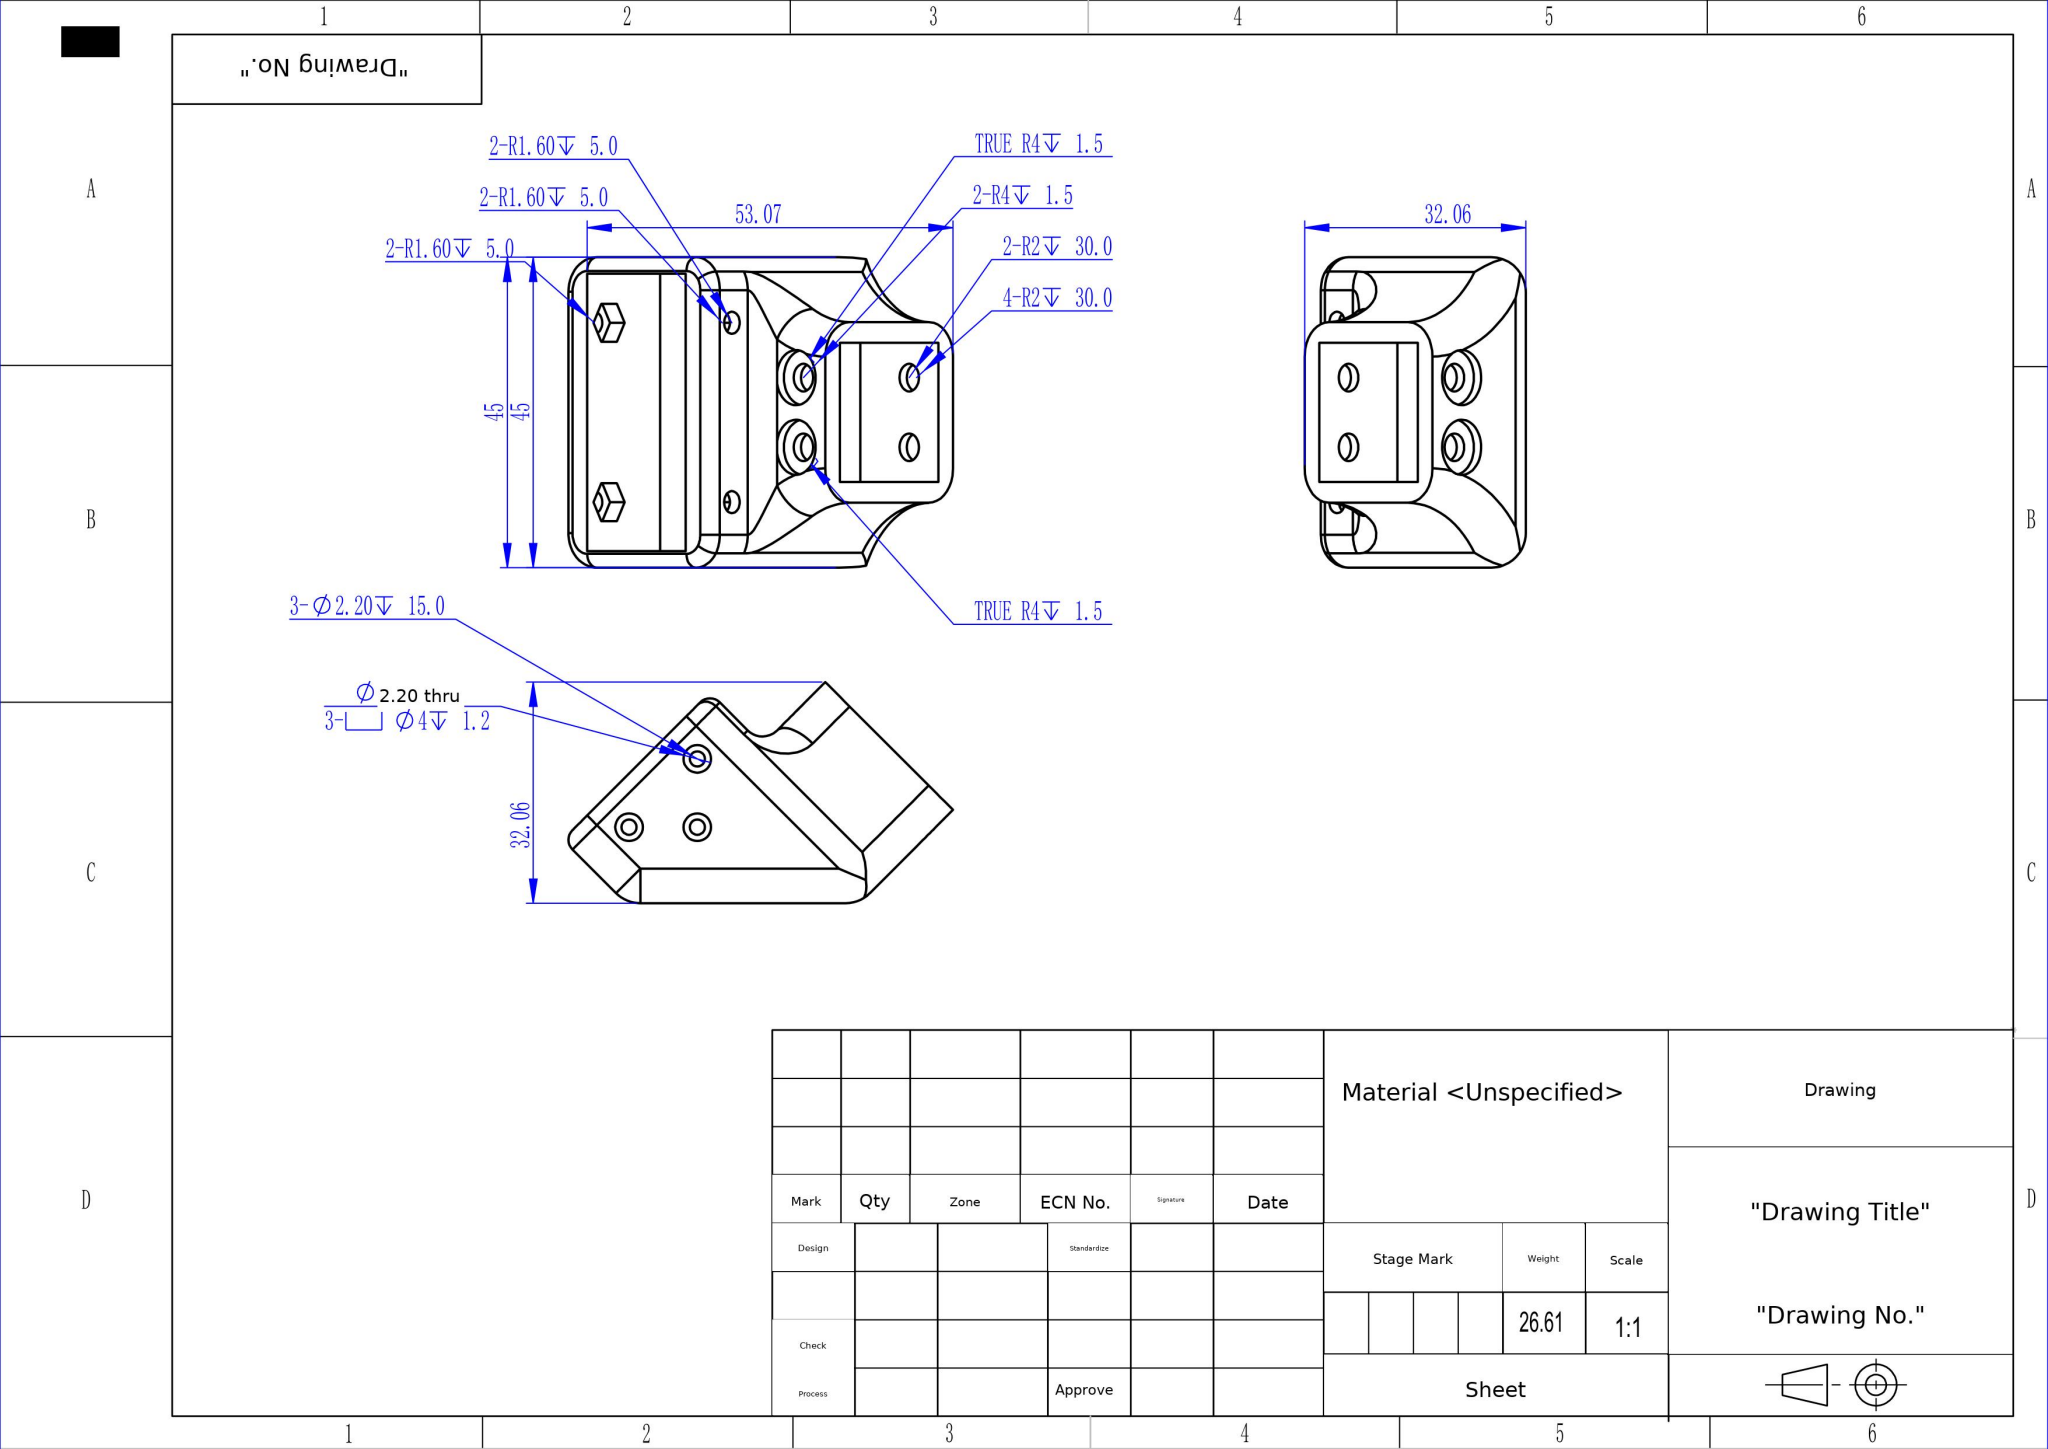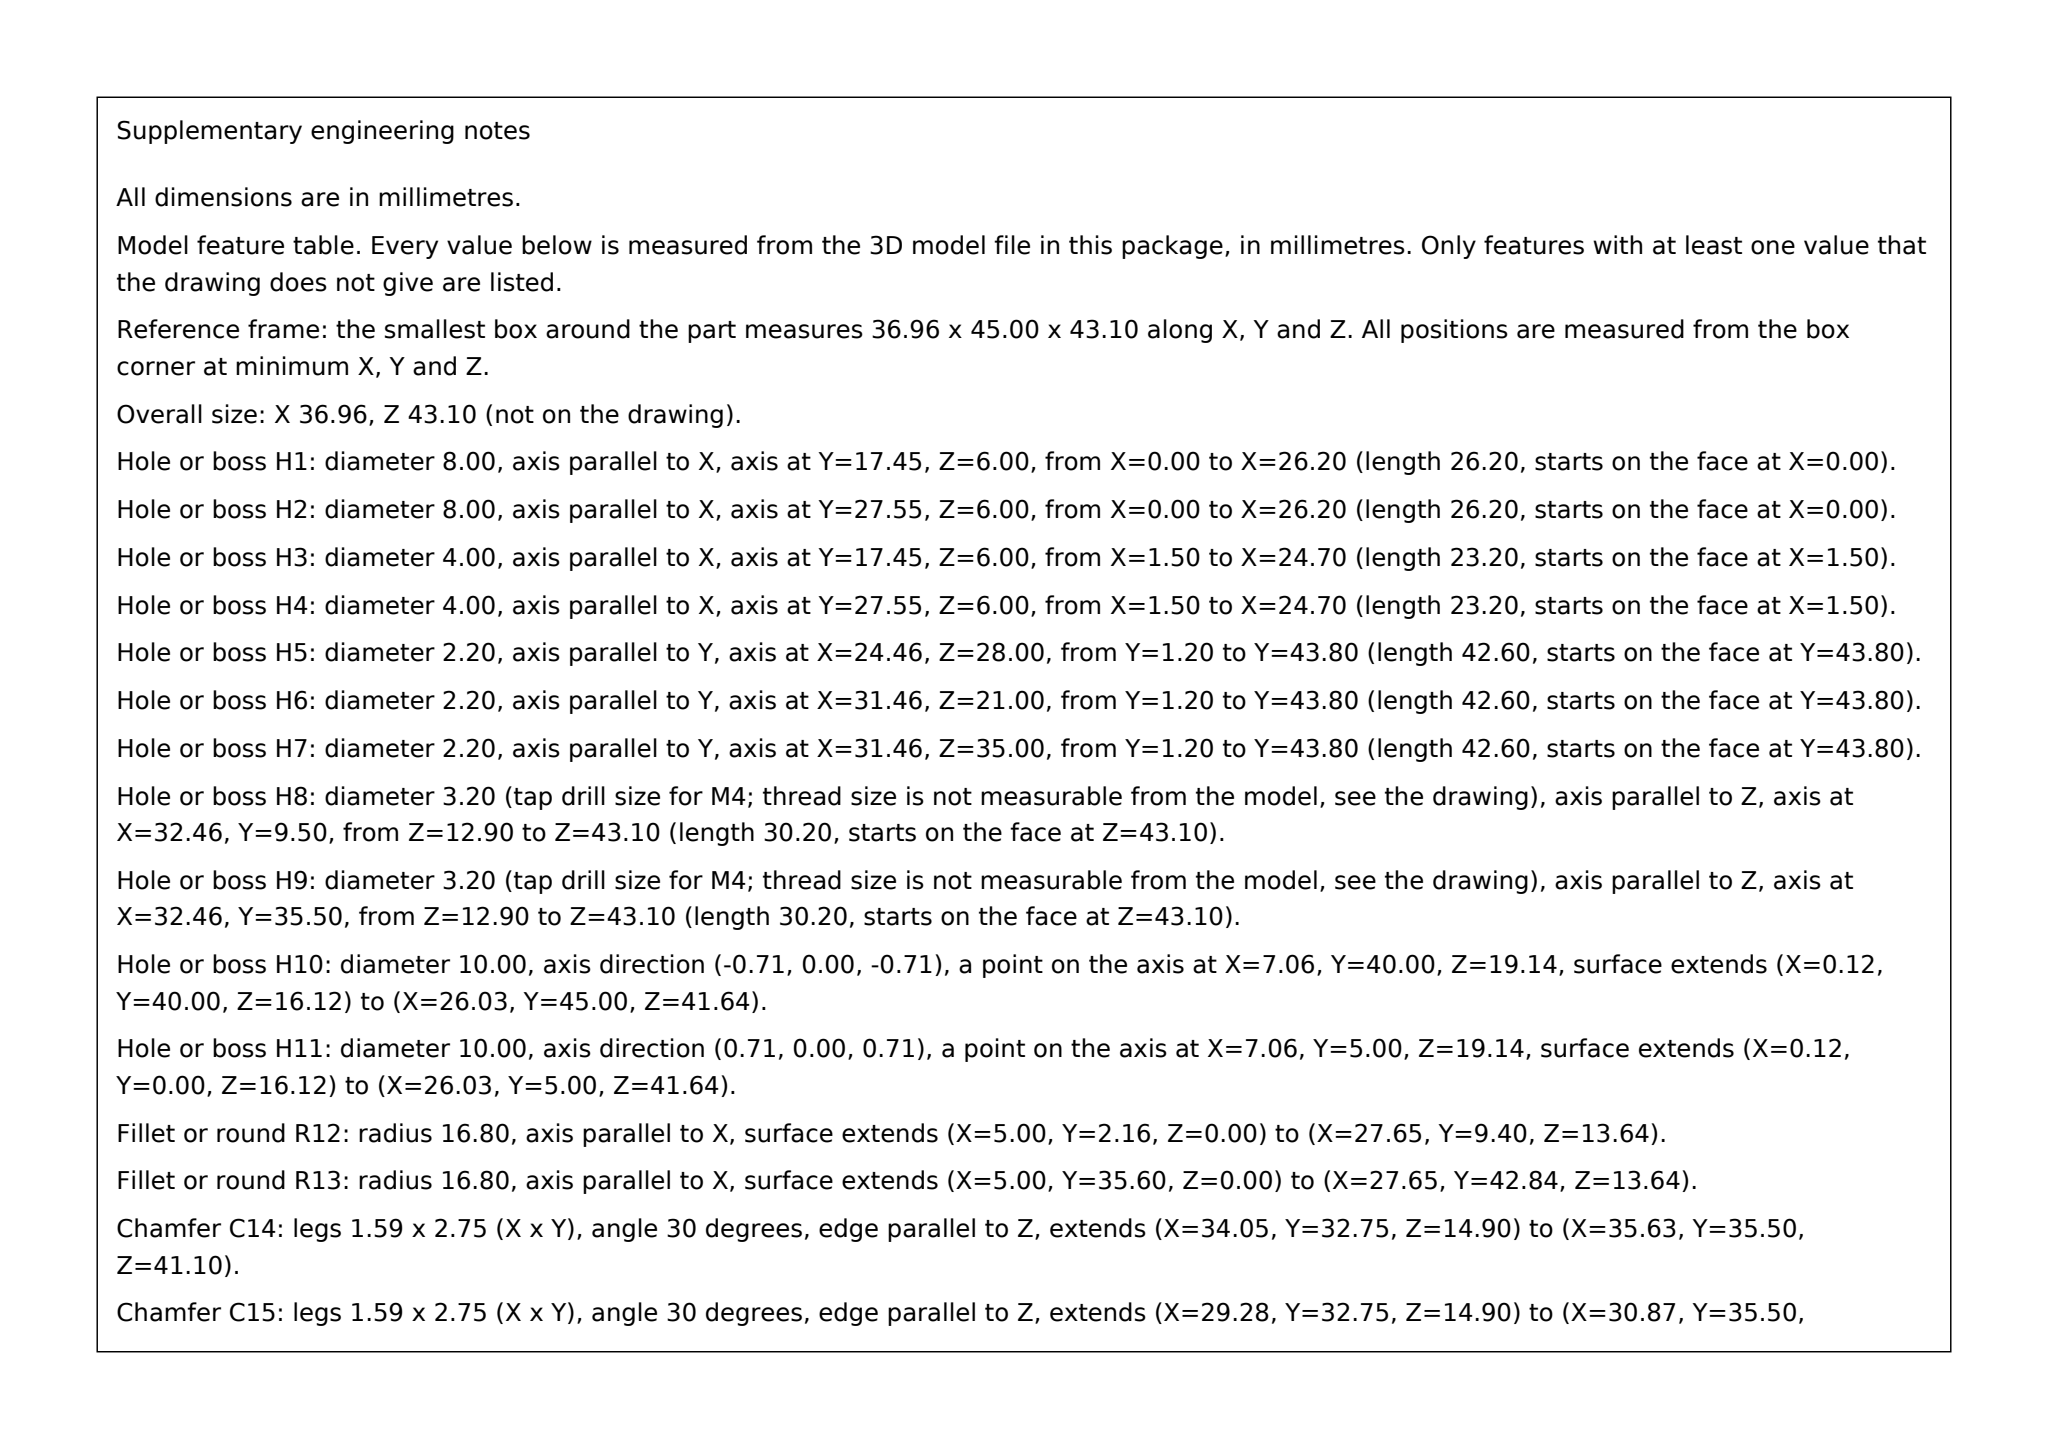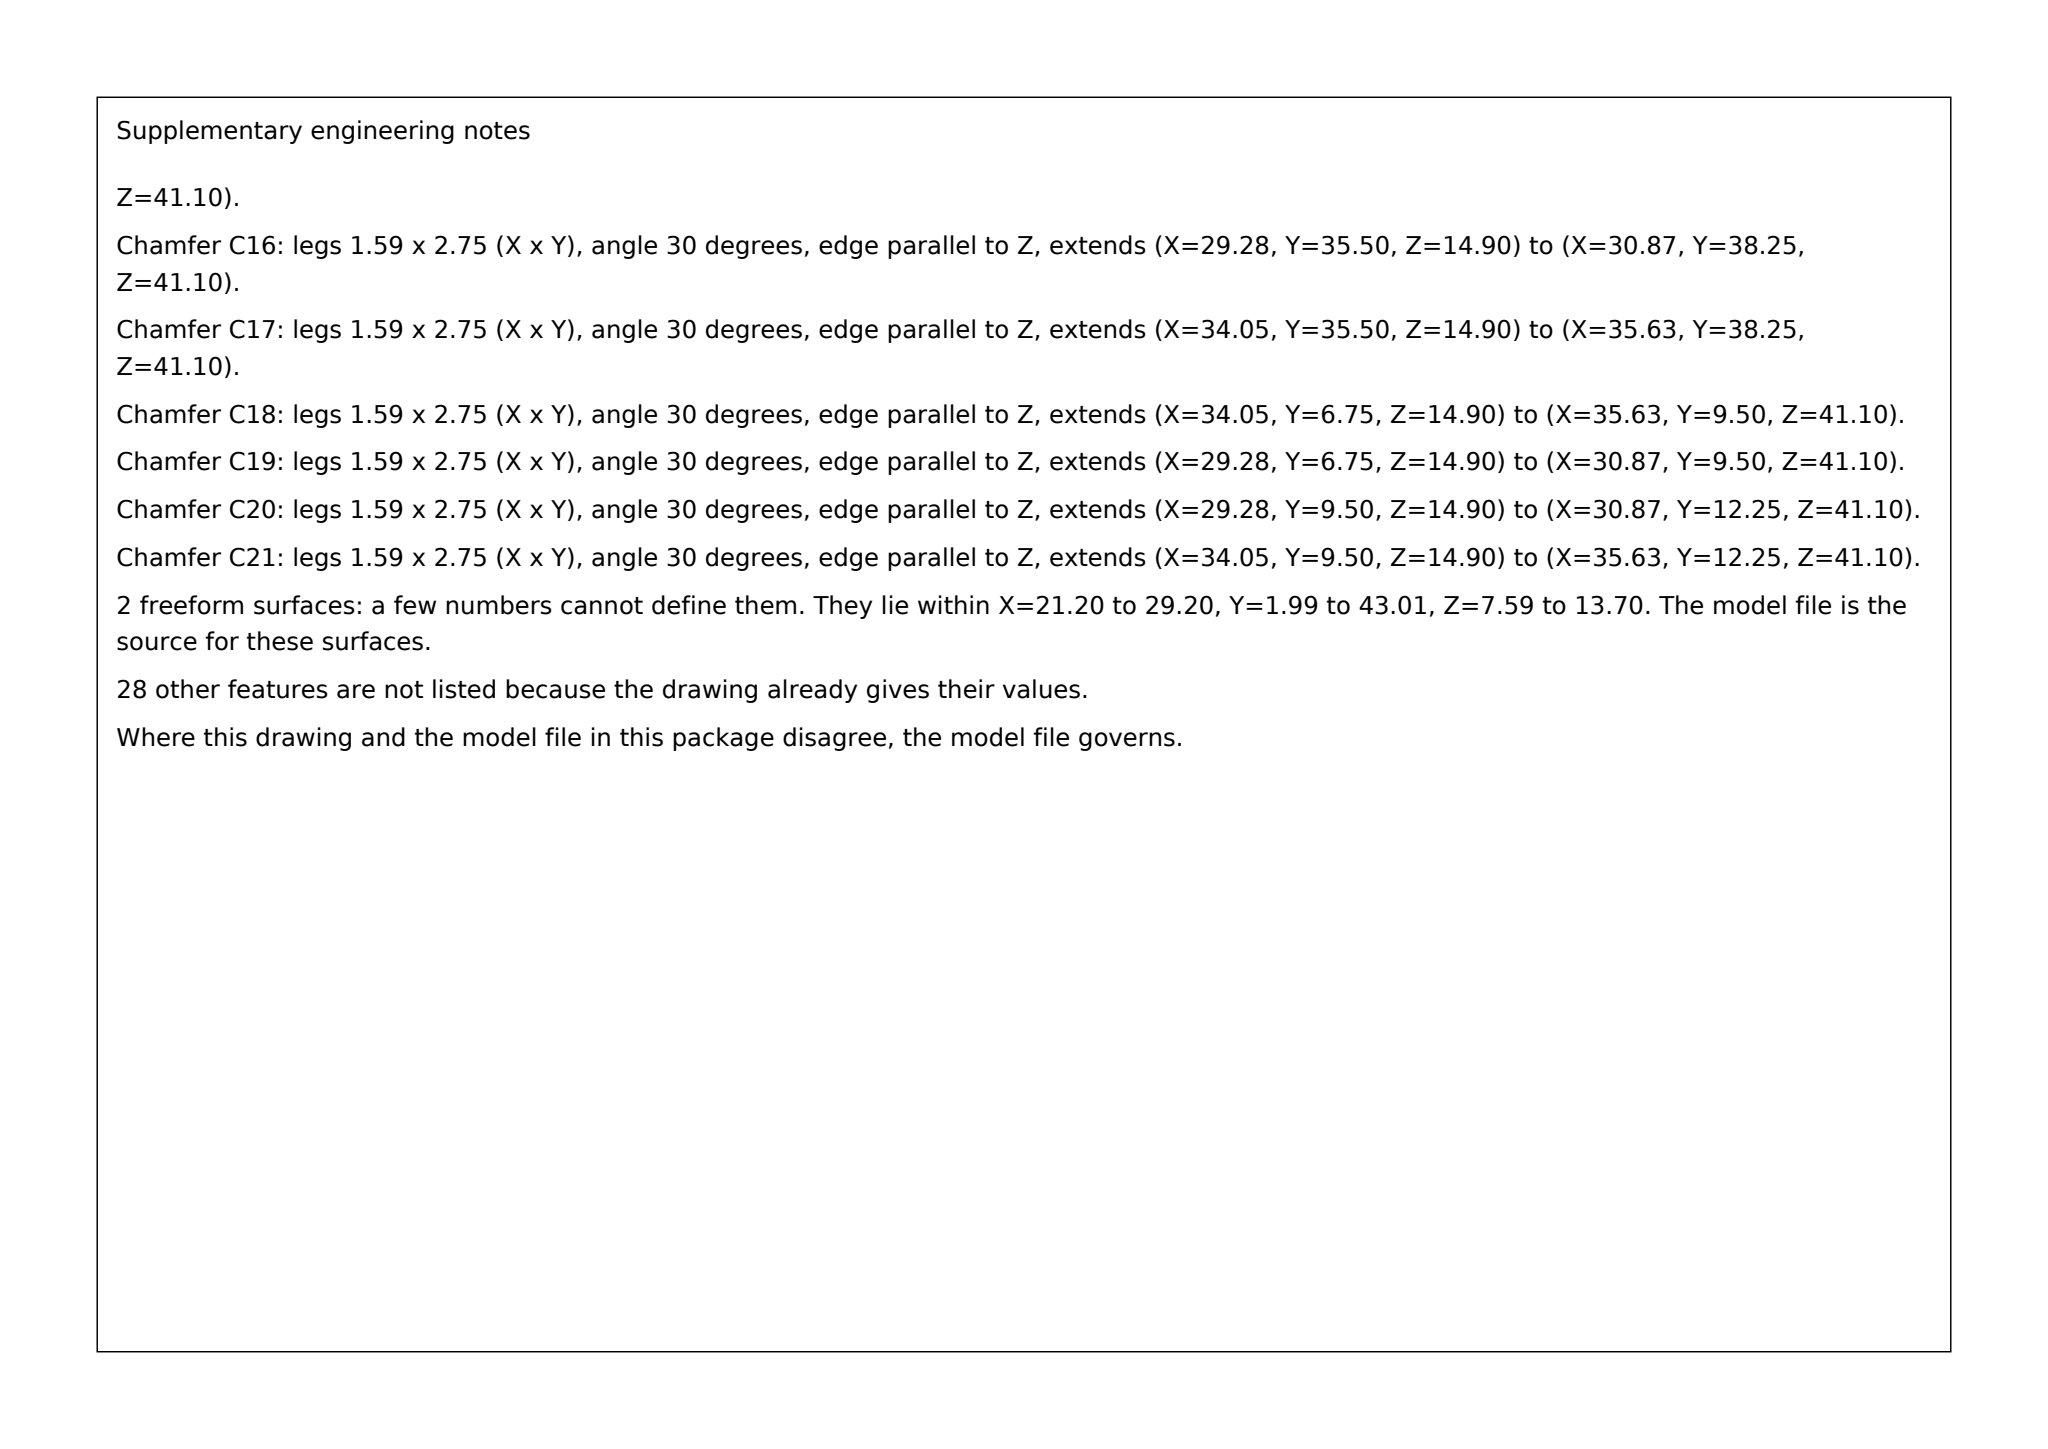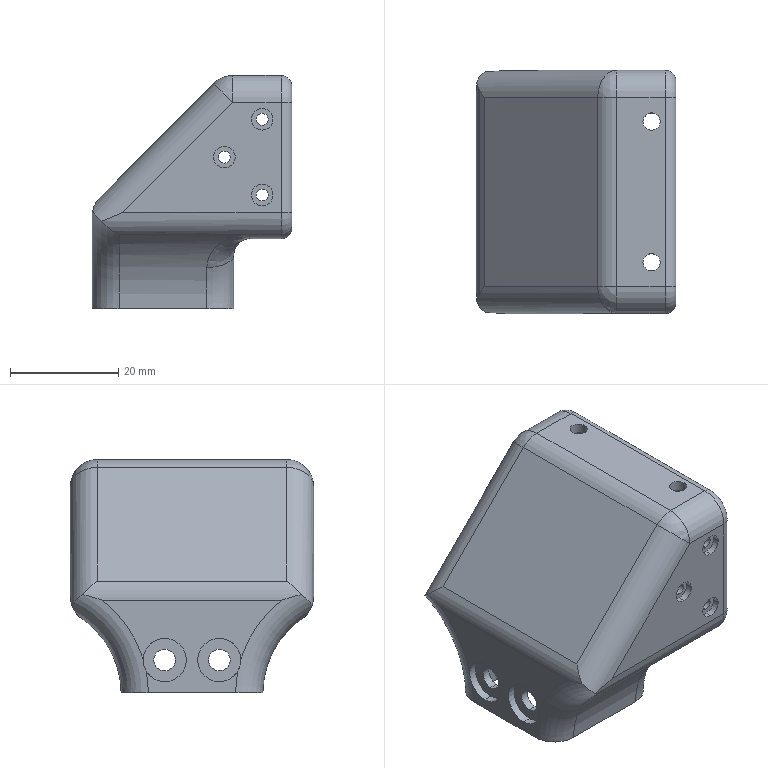Part | SolidWorks | mm | 1 solid | 140 faces | box 36.96 x 45 x 43.1 mm | volume 26613 mm3 | cylinder 65 | plane 61 | torus 10 | spline 2 | sphere 2 | commonest cylinder face diameters 4 x24 2.2 x12 10 x10 8 x8 3.2 x8 33.591 x2 6 x1